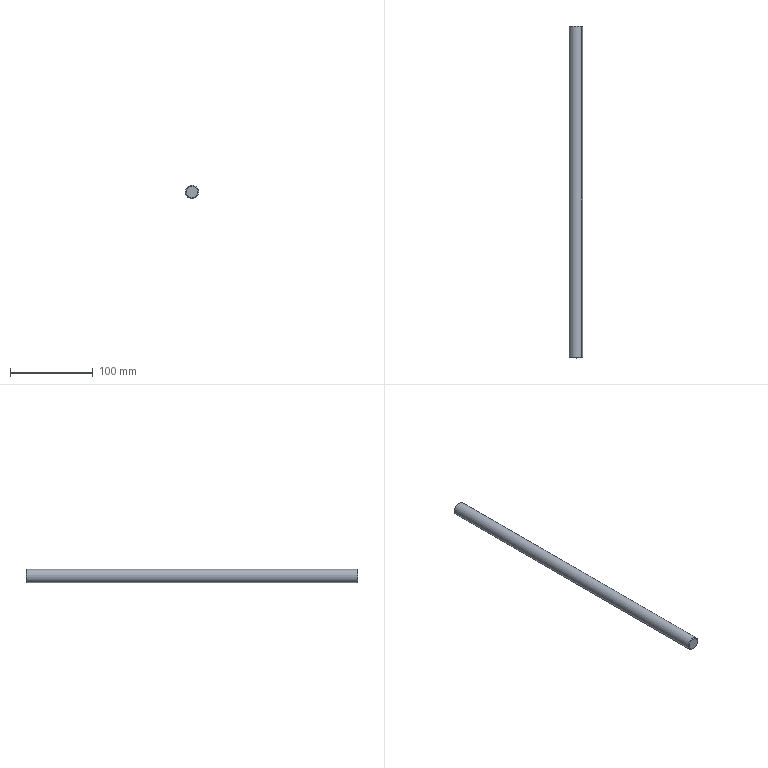Component | SolidWorks | MaterialRod-1 | 1 solid | 8 faces | box 16 x 400 x 16 mm | volume 80377 mm3 | cone 4 | cylinder 2 | plane 2 | commonest cylinder face diameters 16 x2
build123d program:
from build123d import *

# Parameters (mm, degrees)
SKETCH1_R           = 8
BOSS_EXTRUDE1_DEPTH = 200
CHAMFER1_SIZE       = 1


with BuildPart() as part:
    # Sketch1 → Boss-Extrude1 (new, symmetric)
    with BuildSketch(Plane.XY):
        Circle(SKETCH1_R)
    extrude(amount=BOSS_EXTRUDE1_DEPTH, both=True)

    # Chamfer1
    chamfer1_edges = [part.edges().sort_by_distance(p)[0] for p in [
        (-8, 0, -200),
        (-8, 0, 200),
    ]]
    chamfer(chamfer1_edges, length=CHAMFER1_SIZE)


solid = part.part

# Placed as in the assembly
solid = solid.moved(Location((155, 0.04285, -145), (90, 0, 0)))
STEP:
#1=COLOUR_RGB('',0.7922,0.8196,0.9333);
#2=FILL_AREA_STYLE_COLOUR('',#1);
#3=FILL_AREA_STYLE('',(#2));
#4=SURFACE_STYLE_FILL_AREA(#3);
#5=SURFACE_SIDE_STYLE('',(#4));
#6=SURFACE_STYLE_USAGE(.BOTH.,#5);
#7=PRESENTATION_STYLE_ASSIGNMENT((#6));
#8=CARTESIAN_POINT('',(6.324,-7.872,-5.544));
#9=VERTEX_POINT('',#8);
#10=CARTESIAN_POINT('',(5.881,-7.872,-5.873));
#11=VERTEX_POINT('',#10);
#12=CARTESIAN_POINT('',(6.102,-7.872,-5.709));
#13=DIRECTION('',(0.,-1.,0.));
#14=DIRECTION('',(0.8031,0.,0.5958));
#15=AXIS2_PLACEMENT_3D('',#12,#13,#14);
#16=CIRCLE('',#15,0.2756);
#17=EDGE_CURVE('',#9,#11,#16,.T.);
#18=ORIENTED_EDGE('',*,*,#17,.F.);
#19=CARTESIAN_POINT('',(6.355,-7.833,-5.521));
#20=VERTEX_POINT('',#19);
#21=CARTESIAN_POINT('',(6.324,-7.872,-5.544));
#22=DIRECTION('',(0.5679,0.7071,0.4213));
#23=VECTOR('',#22,39.37);
#24=LINE('',#21,#23);
#25=EDGE_CURVE('',#9,#20,#24,.T.);
#26=ORIENTED_EDGE('',*,*,#25,.T.);
#27=CARTESIAN_POINT('',(5.849,-7.833,-5.896));
#28=VERTEX_POINT('',#27);
#29=CARTESIAN_POINT('',(6.102,-7.833,-5.709));
#30=DIRECTION('',(-0.,1.,-0.));
#31=DIRECTION('',(0.8031,0.,0.5958));
#32=AXIS2_PLACEMENT_3D('',#29,#30,#31);
#33=CIRCLE('',#32,0.315);
#34=EDGE_CURVE('',#28,#20,#33,.T.);
#35=ORIENTED_EDGE('',*,*,#34,.F.);
#36=CARTESIAN_POINT('',(5.881,-7.872,-5.873));
#37=DIRECTION('',(-0.5679,0.7071,-0.4213));
#38=VECTOR('',#37,39.37);
#39=LINE('',#36,#38);
#40=EDGE_CURVE('',#11,#28,#39,.T.);
#41=ORIENTED_EDGE('',*,*,#40,.F.);
#42=EDGE_LOOP('',(#18,#26,#35,#41));
#43=FACE_OUTER_BOUND('',#42,.T.);
#44=CARTESIAN_POINT('',(6.102,-7.872,-5.709));
#45=DIRECTION('',(-0.,1.,-0.));
#46=DIRECTION('',(-0.8031,0.,-0.5958));
#47=AXIS2_PLACEMENT_3D('',#44,#45,#46);
#48=CONICAL_SURFACE('',#47,0.2756,0.7854);
#49=ADVANCED_FACE('',(#43),#48,.T.);
#50=CARTESIAN_POINT('',(5.881,7.876,-5.873));
#51=VERTEX_POINT('',#50);
#52=CARTESIAN_POINT('',(6.324,7.876,-5.544));
#53=VERTEX_POINT('',#52);
#54=CARTESIAN_POINT('',(6.102,7.876,-5.709));
#55=DIRECTION('',(-0.,1.,-0.));
#56=DIRECTION('',(0.8031,0.,0.5958));
#57=AXIS2_PLACEMENT_3D('',#54,#55,#56);
#58=CIRCLE('',#57,0.2756);
#59=EDGE_CURVE('',#51,#53,#58,.T.);
#60=ORIENTED_EDGE('',*,*,#59,.F.);
#61=CARTESIAN_POINT('',(5.849,7.836,-5.896));
#62=VERTEX_POINT('',#61);
#63=CARTESIAN_POINT('',(5.849,7.836,-5.896));
#64=DIRECTION('',(-0.5679,-0.7071,-0.4213));
#65=VECTOR('',#64,39.37);
#66=LINE('',#63,#65);
#67=EDGE_CURVE('',#51,#62,#66,.T.);
#68=ORIENTED_EDGE('',*,*,#67,.T.);
#69=CARTESIAN_POINT('',(6.355,7.836,-5.521));
#70=VERTEX_POINT('',#69);
#71=CARTESIAN_POINT('',(6.102,7.836,-5.709));
#72=DIRECTION('',(0.,-1.,0.));
#73=DIRECTION('',(0.8031,0.,0.5958));
#74=AXIS2_PLACEMENT_3D('',#71,#72,#73);
#75=CIRCLE('',#74,0.315);
#76=EDGE_CURVE('',#70,#62,#75,.T.);
#77=ORIENTED_EDGE('',*,*,#76,.F.);
#78=CARTESIAN_POINT('',(6.355,7.836,-5.521));
#79=DIRECTION('',(0.5679,-0.7071,0.4213));
#80=VECTOR('',#79,39.37);
#81=LINE('',#78,#80);
#82=EDGE_CURVE('',#53,#70,#81,.T.);
#83=ORIENTED_EDGE('',*,*,#82,.F.);
#84=EDGE_LOOP('',(#60,#68,#77,#83));
#85=FACE_OUTER_BOUND('',#84,.T.);
#86=CARTESIAN_POINT('',(6.102,7.836,-5.709));
#87=DIRECTION('',(0.,-1.,0.));
#88=DIRECTION('',(0.8031,0.,0.5958));
#89=AXIS2_PLACEMENT_3D('',#86,#87,#88);
#90=CONICAL_SURFACE('',#89,0.315,0.7854);
#91=ADVANCED_FACE('',(#85),#90,.T.);
#92=ORIENTED_EDGE('',*,*,#34,.T.);
#93=CARTESIAN_POINT('',(6.355,-7.872,-5.521));
#94=DIRECTION('',(-0.,1.,-0.));
#95=VECTOR('',#94,39.37);
#96=LINE('',#93,#95);
#97=EDGE_CURVE('',#20,#70,#96,.T.);
#98=ORIENTED_EDGE('',*,*,#97,.T.);
#99=ORIENTED_EDGE('',*,*,#76,.T.);
#100=CARTESIAN_POINT('',(5.849,-7.872,-5.896));
#101=DIRECTION('',(-0.,1.,-0.));
#102=VECTOR('',#101,39.37);
#103=LINE('',#100,#102);
#104=EDGE_CURVE('',#28,#62,#103,.T.);
#105=ORIENTED_EDGE('',*,*,#104,.F.);
#106=EDGE_LOOP('',(#92,#98,#99,#105));
#107=FACE_OUTER_BOUND('',#106,.T.);
#108=CARTESIAN_POINT('',(6.102,-7.872,-5.709));
#109=DIRECTION('',(-0.,1.,-0.));
#110=DIRECTION('',(-0.8031,0.,-0.5958));
#111=AXIS2_PLACEMENT_3D('',#108,#109,#110);
#112=CYLINDRICAL_SURFACE('',#111,0.315);
#113=ADVANCED_FACE('',(#107),#112,.T.);
#114=ORIENTED_EDGE('',*,*,#97,.F.);
#115=CARTESIAN_POINT('',(6.102,-7.833,-5.709));
#116=DIRECTION('',(-0.,1.,-0.));
#117=DIRECTION('',(0.8031,0.,0.5958));
#118=AXIS2_PLACEMENT_3D('',#115,#116,#117);
#119=CIRCLE('',#118,0.315);
#120=EDGE_CURVE('',#20,#28,#119,.T.);
#121=ORIENTED_EDGE('',*,*,#120,.T.);
#122=ORIENTED_EDGE('',*,*,#104,.T.);
#123=CARTESIAN_POINT('',(6.102,7.836,-5.709));
#124=DIRECTION('',(0.,-1.,0.));
#125=DIRECTION('',(0.8031,0.,0.5958));
#126=AXIS2_PLACEMENT_3D('',#123,#124,#125);
#127=CIRCLE('',#126,0.315);
#128=EDGE_CURVE('',#62,#70,#127,.T.);
#129=ORIENTED_EDGE('',*,*,#128,.T.);
#130=EDGE_LOOP('',(#114,#121,#122,#129));
#131=FACE_OUTER_BOUND('',#130,.T.);
#132=CARTESIAN_POINT('',(6.102,-7.872,-5.709));
#133=DIRECTION('',(-0.,1.,-0.));
#134=DIRECTION('',(-0.8031,0.,-0.5958));
#135=AXIS2_PLACEMENT_3D('',#132,#133,#134);
#136=CYLINDRICAL_SURFACE('',#135,0.315);
#137=ADVANCED_FACE('',(#131),#136,.T.);
#138=CARTESIAN_POINT('',(6.102,-7.872,-5.709));
#139=DIRECTION('',(0.,-1.,0.));
#140=DIRECTION('',(0.8031,0.,0.5958));
#141=AXIS2_PLACEMENT_3D('',#138,#139,#140);
#142=CIRCLE('',#141,0.2756);
#143=EDGE_CURVE('',#11,#9,#142,.T.);
#144=ORIENTED_EDGE('',*,*,#143,.T.);
#145=ORIENTED_EDGE('',*,*,#17,.T.);
#146=EDGE_LOOP('',(#144,#145));
#147=FACE_OUTER_BOUND('',#146,.T.);
#148=CARTESIAN_POINT('',(6.102,-7.872,-5.709));
#149=DIRECTION('',(0.,-1.,0.));
#150=DIRECTION('',(0.8031,0.,0.5958));
#151=AXIS2_PLACEMENT_3D('',#148,#149,#150);
#152=PLANE('',#151);
#153=ADVANCED_FACE('',(#147),#152,.T.);
#154=CARTESIAN_POINT('',(6.102,7.876,-5.709));
#155=DIRECTION('',(-0.,1.,-0.));
#156=DIRECTION('',(0.8031,0.,0.5958));
#157=AXIS2_PLACEMENT_3D('',#154,#155,#156);
#158=CIRCLE('',#157,0.2756);
#159=EDGE_CURVE('',#53,#51,#158,.T.);
#160=ORIENTED_EDGE('',*,*,#159,.T.);
#161=ORIENTED_EDGE('',*,*,#59,.T.);
#162=EDGE_LOOP('',(#160,#161));
#163=FACE_OUTER_BOUND('',#162,.T.);
#164=CARTESIAN_POINT('',(6.102,7.876,-5.709));
#165=DIRECTION('',(0.,-1.,0.));
#166=DIRECTION('',(0.8031,0.,0.5958));
#167=AXIS2_PLACEMENT_3D('',#164,#165,#166);
#168=PLANE('',#167);
#169=ADVANCED_FACE('',(#163),#168,.F.);
#170=ORIENTED_EDGE('',*,*,#67,.F.);
#171=ORIENTED_EDGE('',*,*,#159,.F.);
#172=ORIENTED_EDGE('',*,*,#82,.T.);
#173=ORIENTED_EDGE('',*,*,#128,.F.);
#174=EDGE_LOOP('',(#170,#171,#172,#173));
#175=FACE_OUTER_BOUND('',#174,.T.);
#176=CARTESIAN_POINT('',(6.102,7.836,-5.709));
#177=DIRECTION('',(0.,-1.,0.));
#178=DIRECTION('',(0.8031,0.,0.5958));
#179=AXIS2_PLACEMENT_3D('',#176,#177,#178);
#180=CONICAL_SURFACE('',#179,0.315,0.7854);
#181=ADVANCED_FACE('',(#175),#180,.T.);
#182=ORIENTED_EDGE('',*,*,#25,.F.);
#183=ORIENTED_EDGE('',*,*,#143,.F.);
#184=ORIENTED_EDGE('',*,*,#40,.T.);
#185=ORIENTED_EDGE('',*,*,#120,.F.);
#186=EDGE_LOOP('',(#182,#183,#184,#185));
#187=FACE_OUTER_BOUND('',#186,.T.);
#188=CARTESIAN_POINT('',(6.102,-7.872,-5.709));
#189=DIRECTION('',(-0.,1.,-0.));
#190=DIRECTION('',(-0.8031,0.,-0.5958));
#191=AXIS2_PLACEMENT_3D('',#188,#189,#190);
#192=CONICAL_SURFACE('',#191,0.2756,0.7854);
#193=ADVANCED_FACE('',(#187),#192,.T.);
#194=CLOSED_SHELL('',(#49,#91,#113,#137,#153,#169,#181,#193));
#195=MANIFOLD_SOLID_BREP('',#194);
#196=STYLED_ITEM('',(#7),#195);
#197=(LENGTH_UNIT()NAMED_UNIT(*)SI_UNIT($,.METRE.));
#198=LENGTH_MEASURE_WITH_UNIT(LENGTH_MEASURE(0.0254),#197);
#199=DIMENSIONAL_EXPONENTS(1.,0.,0.,0.,0.,0.,0.);
#200=(CONVERSION_BASED_UNIT('',#198)LENGTH_UNIT()NAMED_UNIT(#199));
#201=UNCERTAINTY_MEASURE_WITH_UNIT(LENGTH_MEASURE(0.00001),#200,'','');
#202=(NAMED_UNIT(*)PLANE_ANGLE_UNIT()SI_UNIT($,.RADIAN.));
#203=(NAMED_UNIT(*)SI_UNIT($,.STERADIAN.)SOLID_ANGLE_UNIT());
#204=(GEOMETRIC_REPRESENTATION_CONTEXT(3)GLOBAL_UNCERTAINTY_ASSIGNED_CONTEXT((#201))GLOBAL_UNIT_ASSIGNED_CONTEXT((#200,#202,#203))REPRESENTATION_CONTEXT('',''));
#205=MECHANICAL_DESIGN_GEOMETRIC_PRESENTATION_REPRESENTATION('',(#196),#204);
#206=PRESENTATION_LAYER_ASSIGNMENT('','',(#196));
#207=CARTESIAN_POINT('',(0.,0.,0.));
#208=DIRECTION('',(0.,0.,1.));
#209=DIRECTION('',(1.,0.,0.));
#210=AXIS2_PLACEMENT_3D('',#207,#208,#209);
#211=(LENGTH_UNIT()NAMED_UNIT(*)SI_UNIT($,.METRE.));
#212=LENGTH_MEASURE_WITH_UNIT(LENGTH_MEASURE(0.0254),#211);
#213=DIMENSIONAL_EXPONENTS(1.,0.,0.,0.,0.,0.,0.);
#214=(CONVERSION_BASED_UNIT('',#212)LENGTH_UNIT()NAMED_UNIT(#213));
#215=UNCERTAINTY_MEASURE_WITH_UNIT(LENGTH_MEASURE(0.00001),#214,'','');
#216=(NAMED_UNIT(*)PLANE_ANGLE_UNIT()SI_UNIT($,.RADIAN.));
#217=(NAMED_UNIT(*)SI_UNIT($,.STERADIAN.)SOLID_ANGLE_UNIT());
#218=(GEOMETRIC_REPRESENTATION_CONTEXT(3)GLOBAL_UNCERTAINTY_ASSIGNED_CONTEXT((#215))GLOBAL_UNIT_ASSIGNED_CONTEXT((#214,#216,#217))REPRESENTATION_CONTEXT('',''));
#219=ADVANCED_BREP_SHAPE_REPRESENTATION('',(#195,#210),#218);